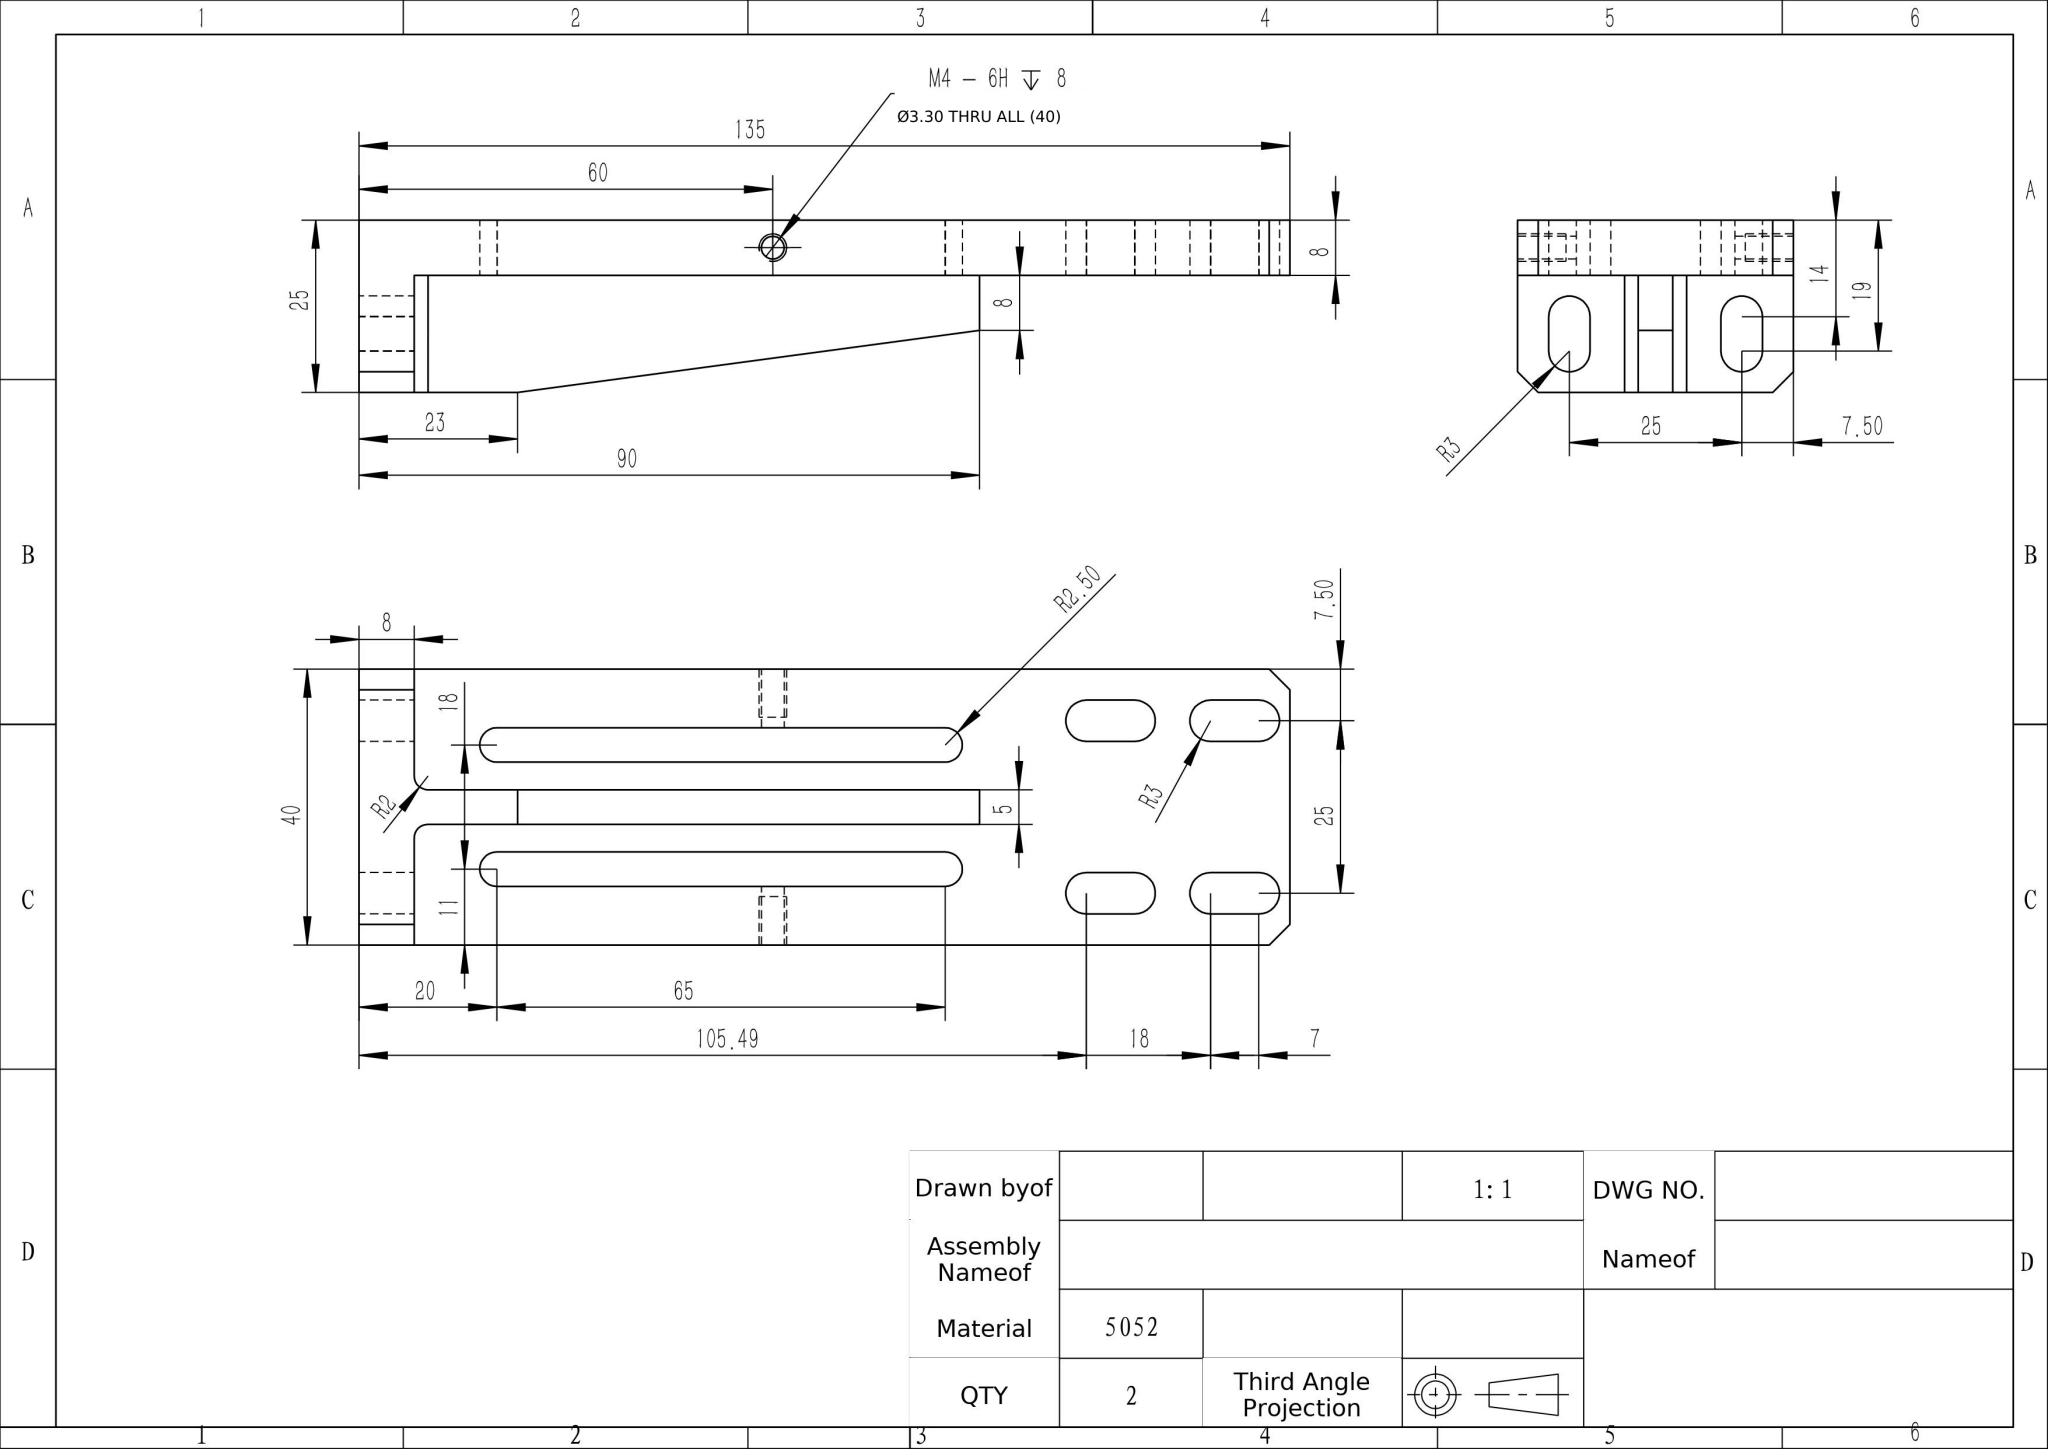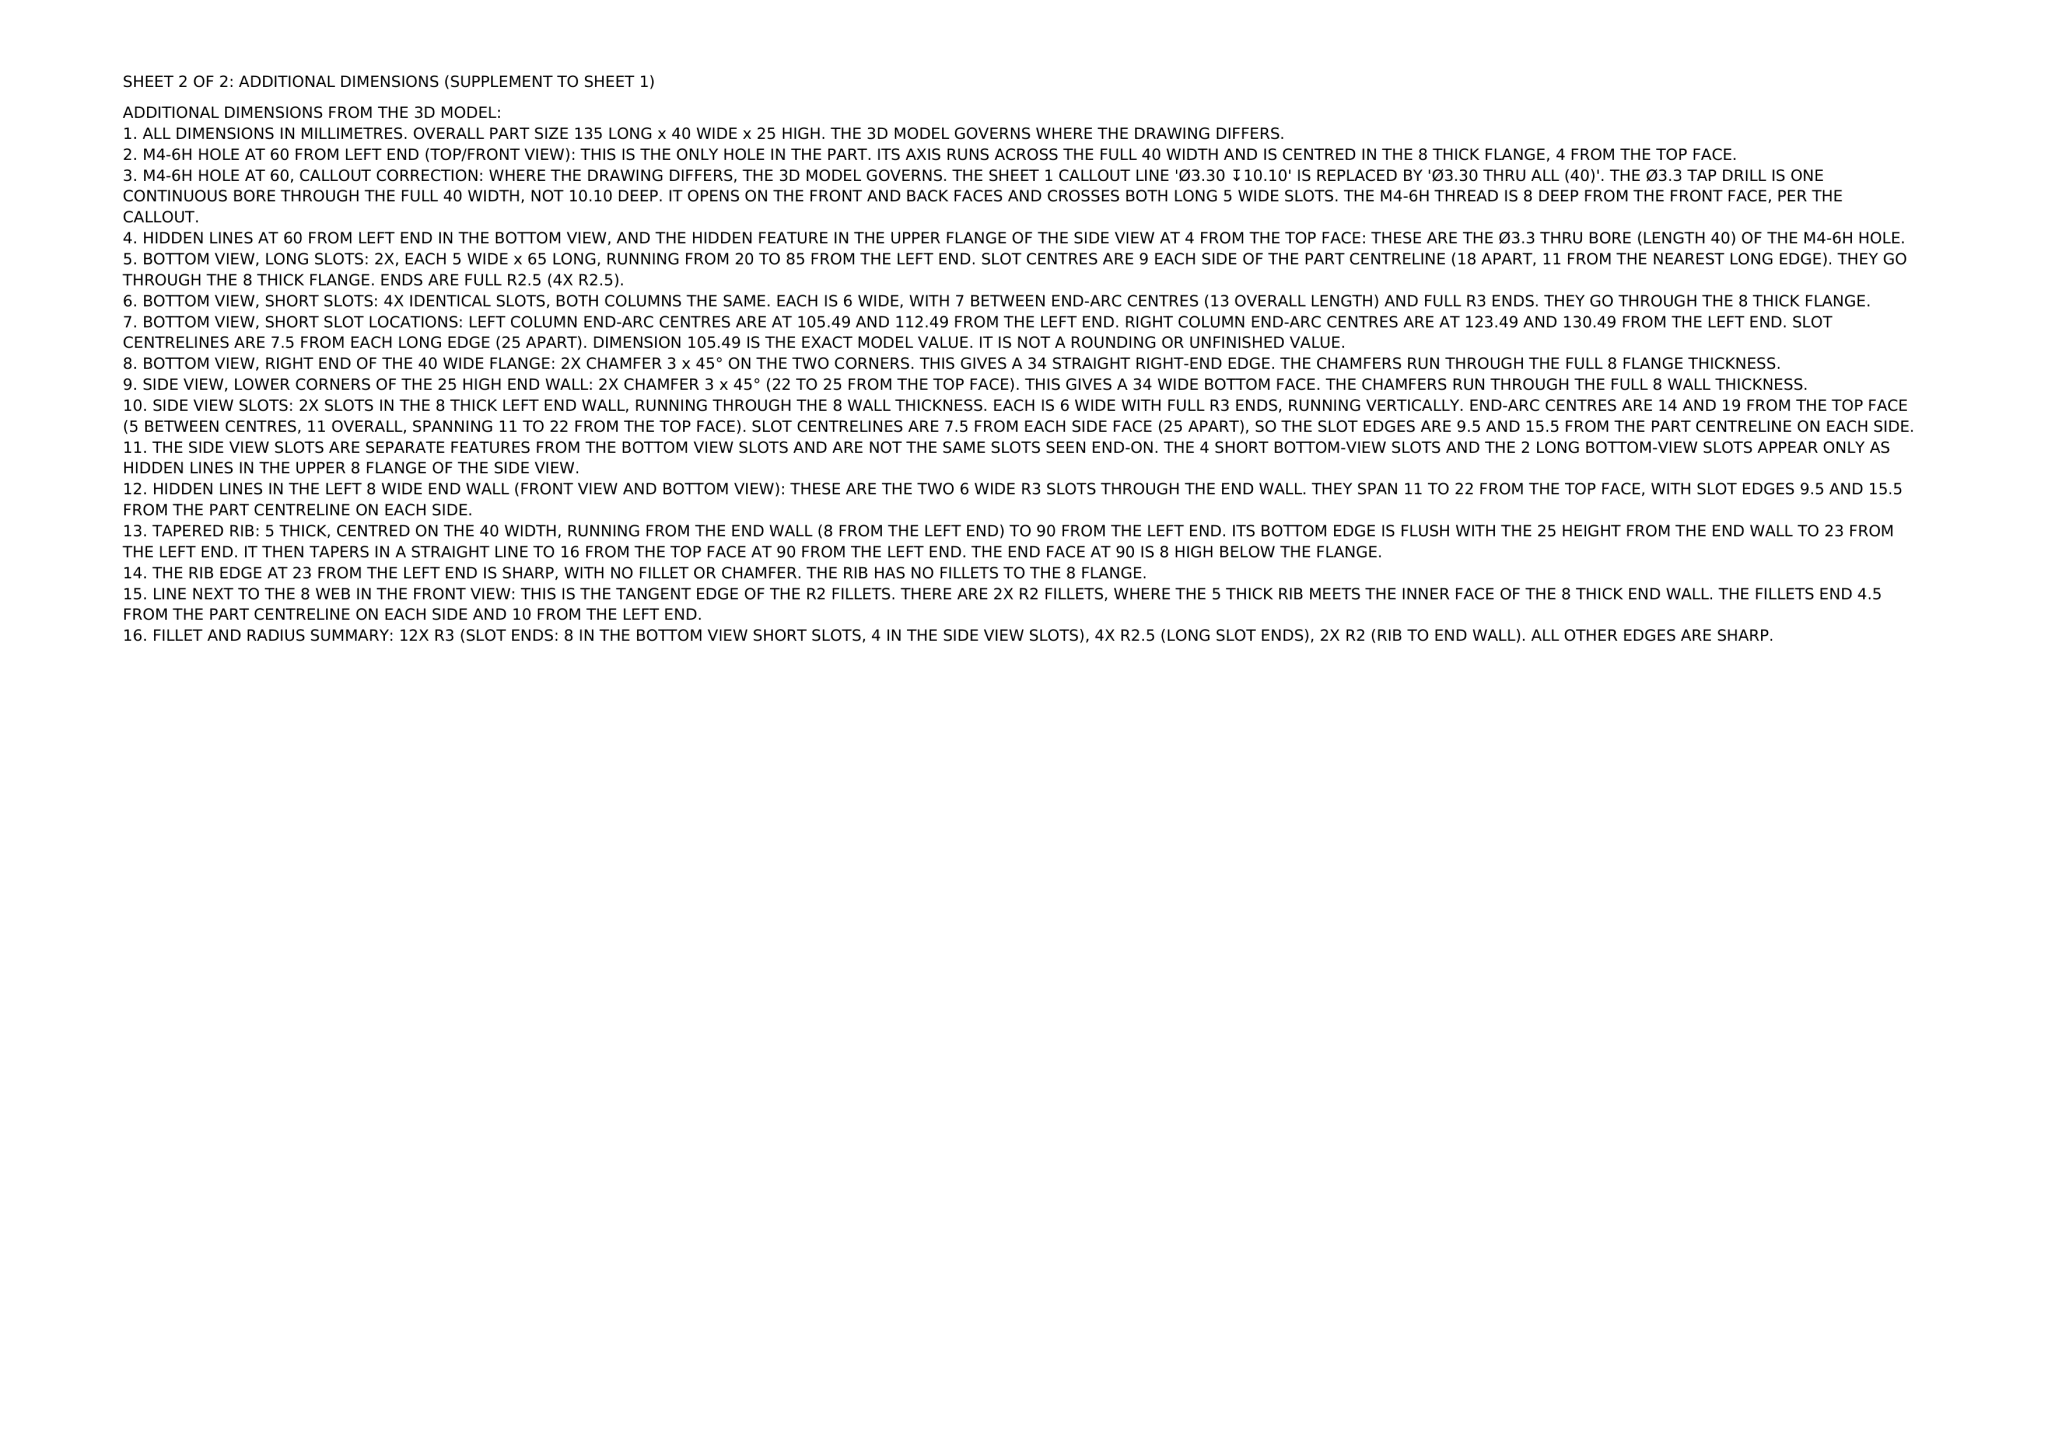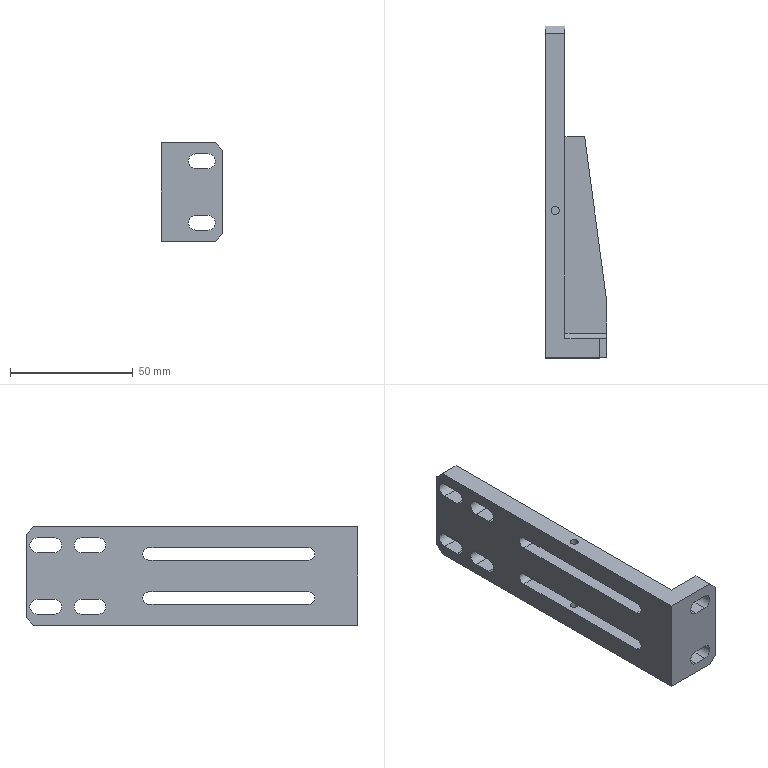Part | NX | mm | 1 solid | 57 faces | box 25 x 135 x 40 mm | volume 45147 mm3 | plane 33 | cylinder 24 | commonest cylinder face diameters 6 x14 3.3 x4 5 x4 4 x2